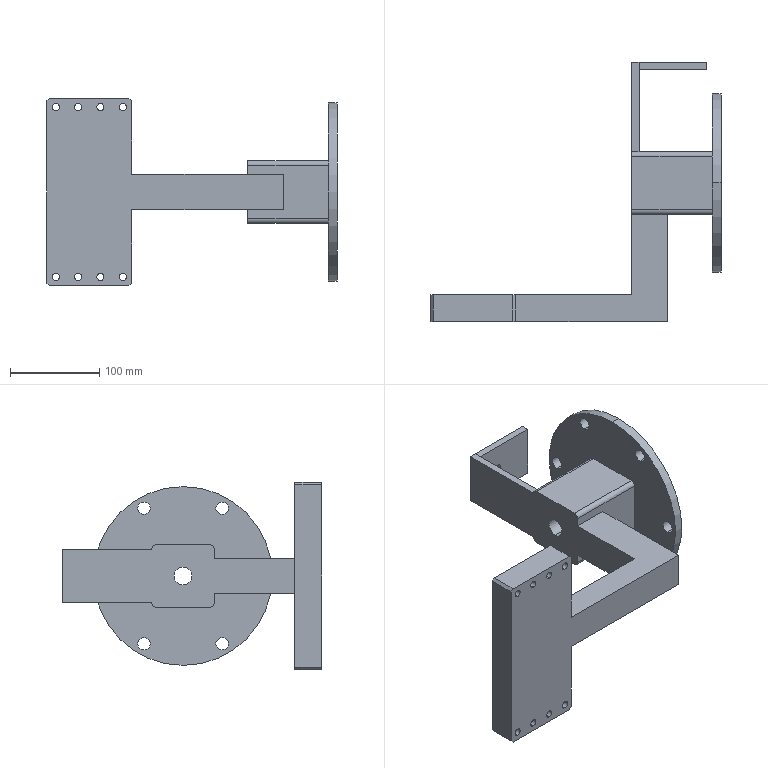Component | SolidWorks | Arm4-1 | 1 solid | 74 faces | box 325 x 290 x 210 mm | volume 1653865 mm3 | cylinder 42 | plane 32 | commonest cylinder face diameters 8 x16 14 x12 10 x8 20 x2 60 x2 200 x2
build123d program:
from build123d import *

# Parameters (mm, degrees)
SKETCH1_W            = 130
SKETCH1_H            = 30
BOSS_EXTRUDE1_DEPTH  = 40
BOSS_EXTRUDE2_DEPTH  = 40
SKETCH20_W           = 90
SKETCH20_H           = 70
BOSS_EXTRUDE8_DEPTH  = 15
SKETCH21_W           = 90
SKETCH21_H           = 70
BOSS_EXTRUDE9_DEPTH  = 15
FILLET1_R            = 5
SKETCH23_R           = 100
BOSS_EXTRUDE12_DEPTH = 10
SKETCH28_R           = 30
CUT_EXTRUDE13_DEPTH  = 30
CUT_EXTRUDE14_REACH  = 343.906
SKETCH31_R           = 10
CUT_EXTRUDE15_REACH  = 362.278
SKETCH33_R           = 7
CIRPATTERN2_COUNT    = 6
BOSS_EXTRUDE13_DEPTH = 30
SKETCH35_R           = 4
CUT_EXTRUDE16_DEPTH  = 346.181
CHAMFER1_SIZE        = 3
SKETCH36_W           = 8
SKETCH36_H           = 60
BOSS_EXTRUDE14_DEPTH = 100
BOSS_EXTRUDE15_DEPTH = 75
CUT_EXTRUDE17_REACH  = 392.672
SKETCH38_R           = 5


with BuildPart() as part:
    # Sketch1 → Boss-Extrude1 (new body)
    with BuildSketch(Plane.XY):
        with Locations((65, 10)):
            Rectangle(SKETCH1_W, SKETCH1_H)
    extrude(amount=BOSS_EXTRUDE1_DEPTH)

    # Sketch11 → Boss-Extrude2 (add)
    with BuildSketch(Plane.XY.offset(40)):
        Polygon((130, -5), (130, 185), (220, 185), (220, 115), (170, 115), (170, -5), align=None)
    extrude(amount=-BOSS_EXTRUDE2_DEPTH)

    # Sketch20 → Boss-Extrude8 (add)
    with BuildSketch(Plane.XY.offset(40)):
        with Locations((175, 150)):
            Rectangle(SKETCH20_W, SKETCH20_H)
    extrude(amount=BOSS_EXTRUDE8_DEPTH)

    # Sketch21 → Boss-Extrude9 (add)
    with BuildSketch(Plane(origin=(0, 0, 0), x_dir=(-1, 0, 0), z_dir=(0, 0, -1))):
        with Locations((-175, 150)):
            Rectangle(SKETCH21_W, SKETCH21_H)
    extrude(amount=BOSS_EXTRUDE9_DEPTH)

    # Fillet1
    fillet1_edges = [part.edges().sort_by_distance(p)[0] for p in [
        (175, 115, 55),
        (175, 115, -15),
        (175, 185, 55),
        (175, 185, -15),
    ]]
    fillet(fillet1_edges, radius=FILLET1_R)

    # Sketch23 → Boss-Extrude12 (add)
    with BuildSketch(Plane(origin=(220, 0, 0), x_dir=(0, 0, -1), z_dir=(1, 0, 0))):
        with Locations((-20, 150)):
            Circle(SKETCH23_R)
    extrude(amount=BOSS_EXTRUDE12_DEPTH)

    # Sketch28 → Cut-Extrude13 (cut)
    with BuildSketch(Plane(origin=(230, 0, 0), x_dir=(0, 0, -1), z_dir=(1, 0, 0))):
        with Locations((-20, 150)):
            Circle(SKETCH28_R)
    extrude(amount=-CUT_EXTRUDE13_DEPTH, mode=Mode.SUBTRACT)

    # Sketch31 → Cut-Extrude14 (cut, up to next)
    with BuildSketch(Plane(origin=(200, 0, 0), x_dir=(0, 0, -1), z_dir=(1, 0, 0)), mode=Mode.PRIVATE) as cut_extrude14_sk1:
        with Locations((-20, 150)):
            Circle(SKETCH31_R)
    cut_extrude14_tool1 = extrude(cut_extrude14_sk1.sketch, amount=-CUT_EXTRUDE14_REACH, mode=Mode.PRIVATE) & part.part
    add(cut_extrude14_tool1.solids().sort_by_distance((200, 150, 20))[0], mode=Mode.SUBTRACT)

    # Sketch33 → Cut-Extrude15 (cut, up to next)
    with BuildSketch(Plane(origin=(230, 0, 0), x_dir=(0, 0, -1), z_dir=(1, 0, 0)), mode=Mode.PRIVATE) as cut_extrude15_sk1:
        with Locations((-20, 237.5)):
            Circle(SKETCH33_R)
    cut_extrude15_tool1 = extrude(cut_extrude15_sk1.sketch, amount=-CUT_EXTRUDE15_REACH, mode=Mode.PRIVATE) & part.part
    cut_extrude15 = cut_extrude15_tool1.solids().sort_by_distance((230, 237.5, 20))[0]
    add(cut_extrude15, mode=Mode.SUBTRACT)

    # CirPattern2: Cut-Extrude15 ×6 about axis
    cirpattern2_axis = Axis((0, 150, 20), (1, 0, 0))
    for i in range(1, CIRPATTERN2_COUNT):
        add(cut_extrude15.rotate(cirpattern2_axis, i * 360 / CIRPATTERN2_COUNT), mode=Mode.SUBTRACT)

    # Sketch34 → Boss-Extrude13 (add)
    with BuildSketch(Plane.XZ.offset(5)):
        Polygon((0, -85), (0, 125), (-95, 125), (-95, 20), (-95, -85), align=None)
    extrude(amount=-BOSS_EXTRUDE13_DEPTH)

    # Sketch35 → Cut-Extrude16 (cut, through all)
    with BuildSketch(Plane(origin=(0, 25, 0), x_dir=(1, 0, 0), z_dir=(0, 1, 0))):
        with Locations(Location((-85, 75, 0), (0, 0, 270))):
            Circle(SKETCH35_R)
        with Locations(Location((-60, 75, 0), (0, 0, 270))):
            Circle(SKETCH35_R)
        with Locations(Location((-35, 75, 0), (0, 0, 270))):
            Circle(SKETCH35_R)
        with Locations(Location((-10, 75, 0), (0, 0, 270))):
            Circle(SKETCH35_R)
        with Locations(Location((-10, -115, 0), (0, 0, 180))):
            Circle(SKETCH35_R)
        with Locations(Location((-35, -115, 0), (0, 0, 180))):
            Circle(SKETCH35_R)
        with Locations(Location((-60, -115, 0), (0, 0, 180))):
            Circle(SKETCH35_R)
        with Locations(Location((-85, -115, 0), (0, 0, 180))):
            Circle(SKETCH35_R)
    extrude(amount=-CUT_EXTRUDE16_DEPTH, mode=Mode.SUBTRACT)

    # Chamfer1
    chamfer1_edges = [part.edges().sort_by_distance(p)[0] for p in [
        (0, 10, 125),
        (-95, 10, 125),
        (0, 10, -85),
        (-95, 10, -85),
    ]]
    chamfer(chamfer1_edges, length=CHAMFER1_SIZE)

    # Sketch36 → Boss-Extrude14 (add)
    with BuildSketch(Plane(origin=(0, 185, 0), x_dir=(1, 0, 0), z_dir=(0, 1, 0))):
        with Locations((134, -20)):
            Rectangle(SKETCH36_W, SKETCH36_H)
    extrude(amount=BOSS_EXTRUDE14_DEPTH)

    # Sketch37 → Boss-Extrude15 (add)
    with BuildSketch(Plane(origin=(138, 0, 0), x_dir=(0, 0, -1), z_dir=(1, 0, 0))):
        Polygon((-50, 285), (-50.04, 285), (-50.04, 277), (10.04, 277), (10.04, 285), (10, 285), align=None)
    extrude(amount=BOSS_EXTRUDE15_DEPTH)

    # Sketch38 → Cut-Extrude17 (cut, up to next)
    with BuildSketch(Plane(origin=(0, 285, 0), x_dir=(1, 0, 0), z_dir=(0, 1, 0)), mode=Mode.PRIVATE) as cut_extrude17_sk1:
        with Locations(Location((145, -20, 0), (0, 0, 270))):
            Circle(SKETCH38_R)
    cut_extrude17_tool1 = extrude(cut_extrude17_sk1.sketch, amount=-CUT_EXTRUDE17_REACH, mode=Mode.PRIVATE) & part.part
    # Sketch38 → Cut-Extrude17 (cut, up to next)
    with BuildSketch(Plane(origin=(0, 285, 0), x_dir=(1, 0, 0), z_dir=(0, 1, 0)), mode=Mode.PRIVATE) as cut_extrude17_sk2:
        with Locations(Location((165.2, -20, 0), (0, 0, 270))):
            Circle(SKETCH38_R)
    cut_extrude17_tool2 = extrude(cut_extrude17_sk2.sketch, amount=-CUT_EXTRUDE17_REACH, mode=Mode.PRIVATE) & part.part
    add(cut_extrude17_tool1.solids().sort_by_distance((145, 285, 20))[0], mode=Mode.SUBTRACT)
    add(cut_extrude17_tool2.solids().sort_by_distance((165.2, 285, 20))[0], mode=Mode.SUBTRACT)


solid = part.part

# Placed as in the assembly
solid = solid.moved(Location((-114.359, -79.337, -20), (0, 0, 0)))